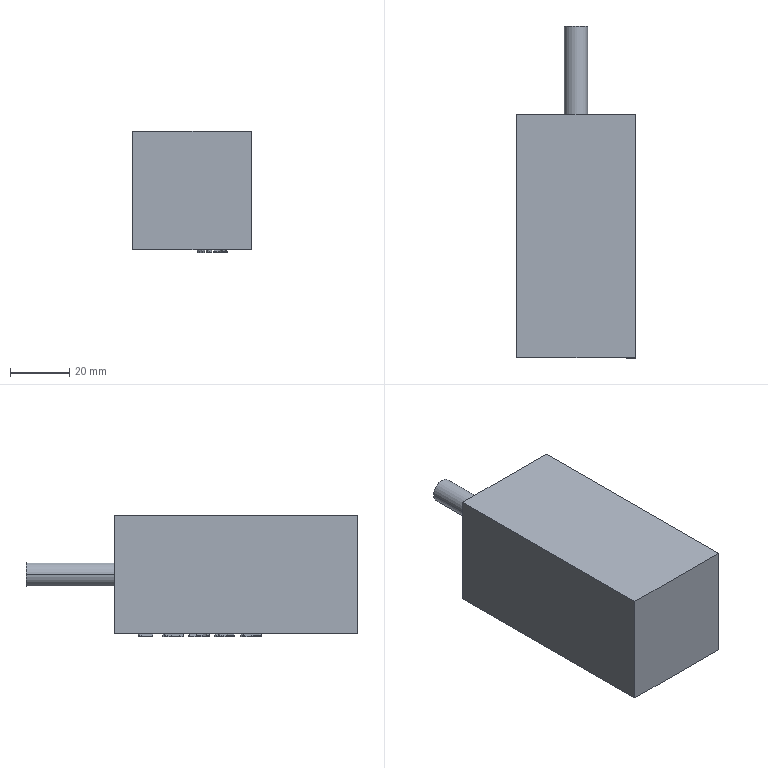Component | SolidWorks | Y-AxisAssembly-1_100WServoMotor-1 | 1 solid | 426 faces | box 40 x 112.4 x 41 mm | volume 133380 mm3 | plane 304 | spline 120 | cylinder 2 | commonest cylinder face diameters 8 x2